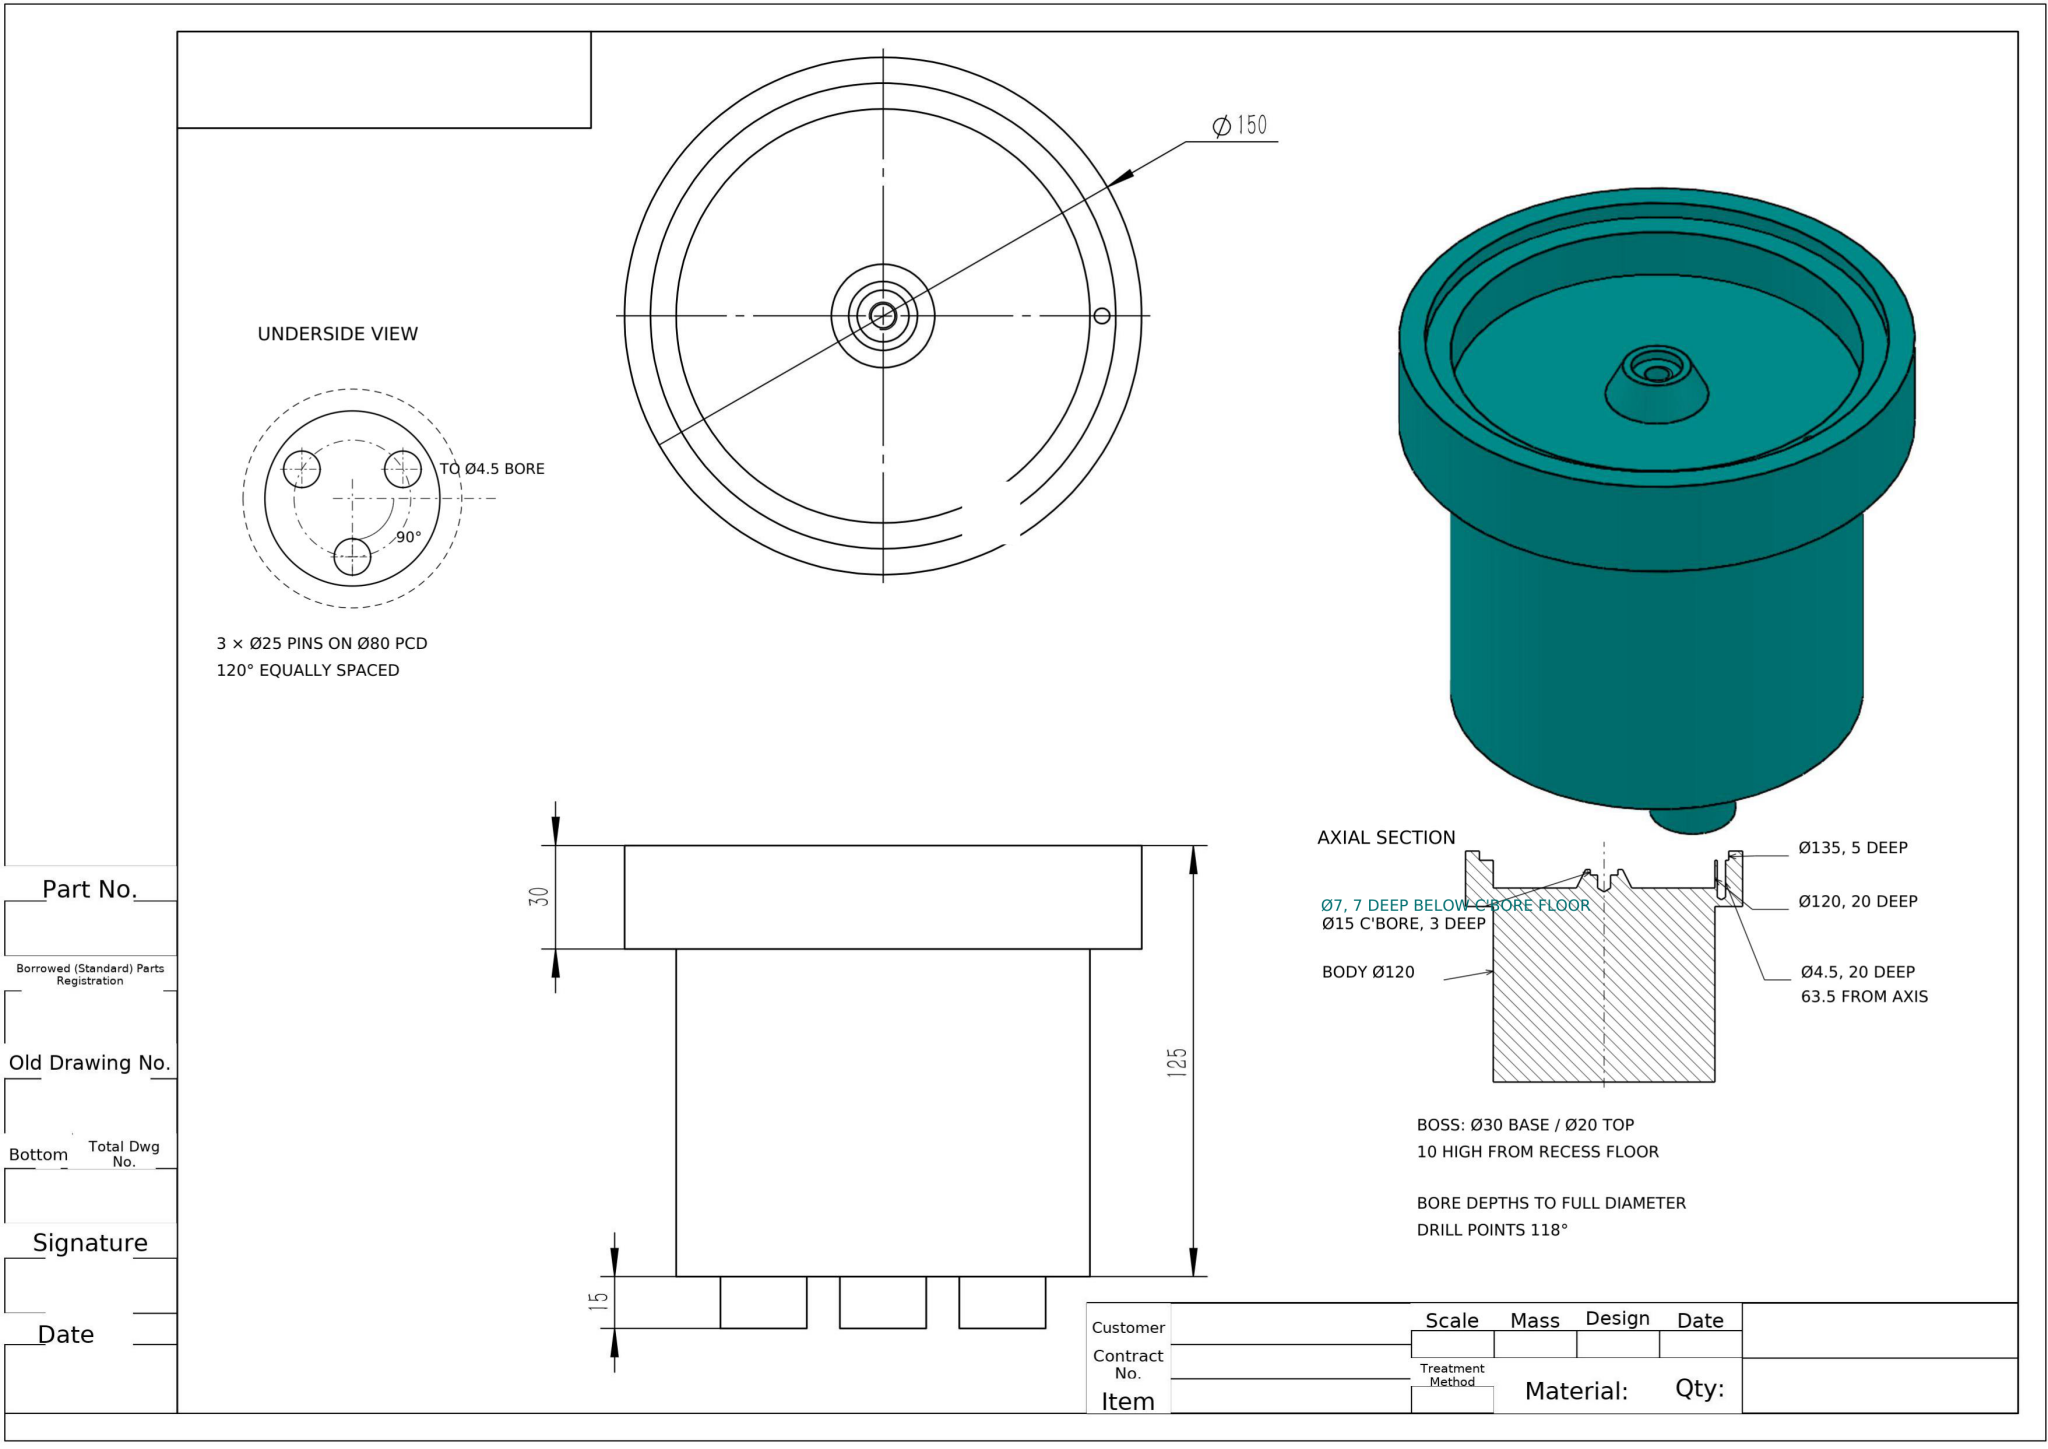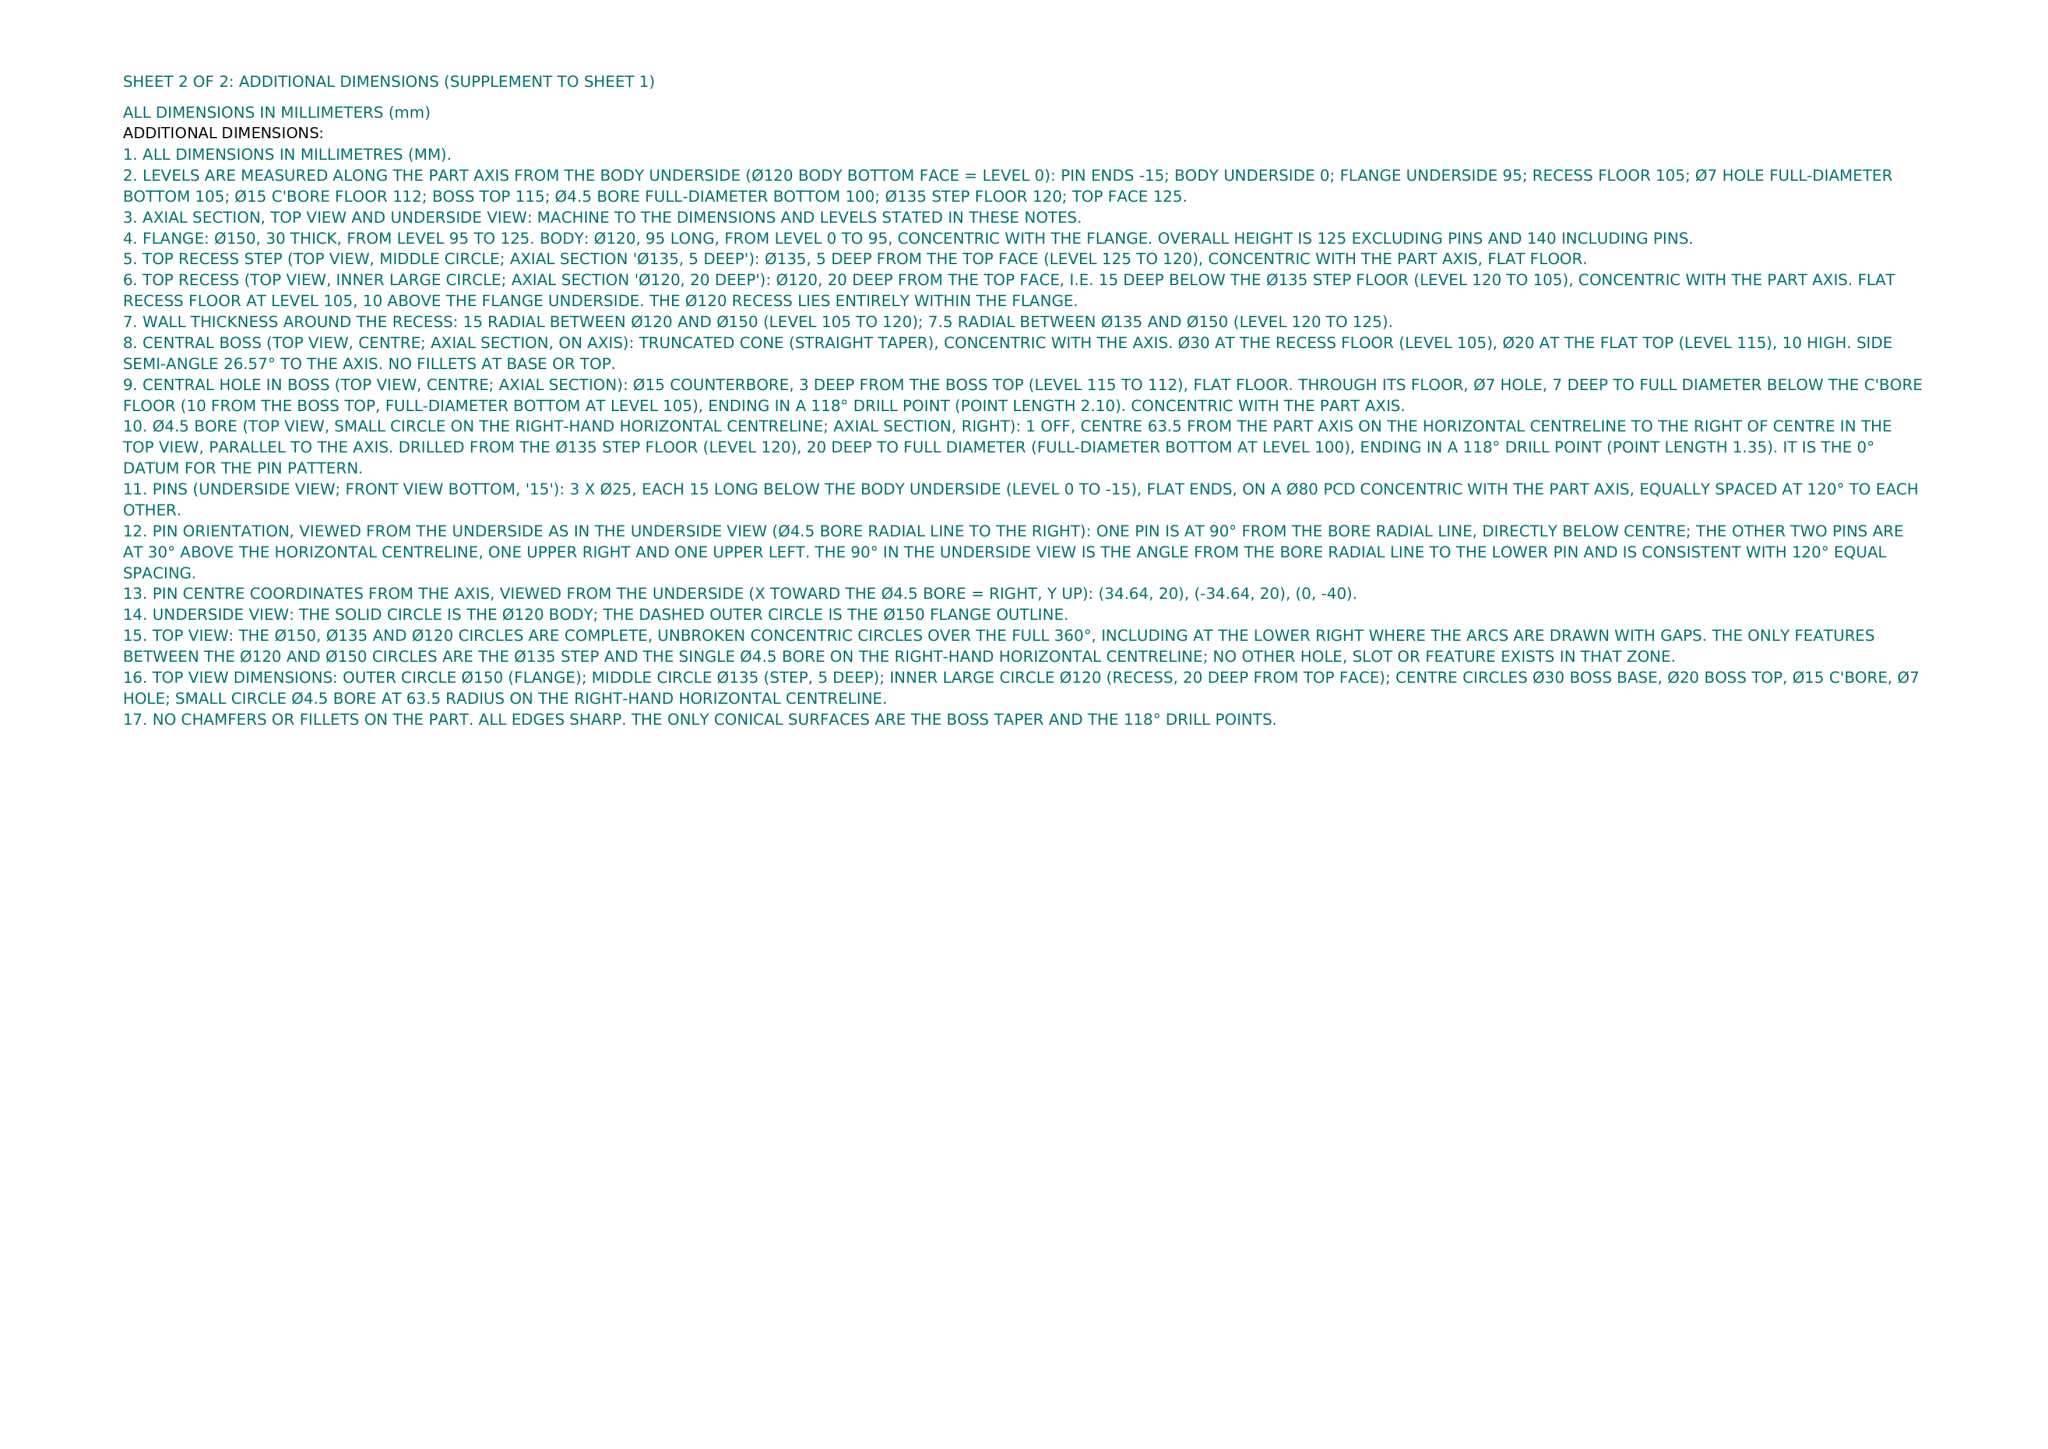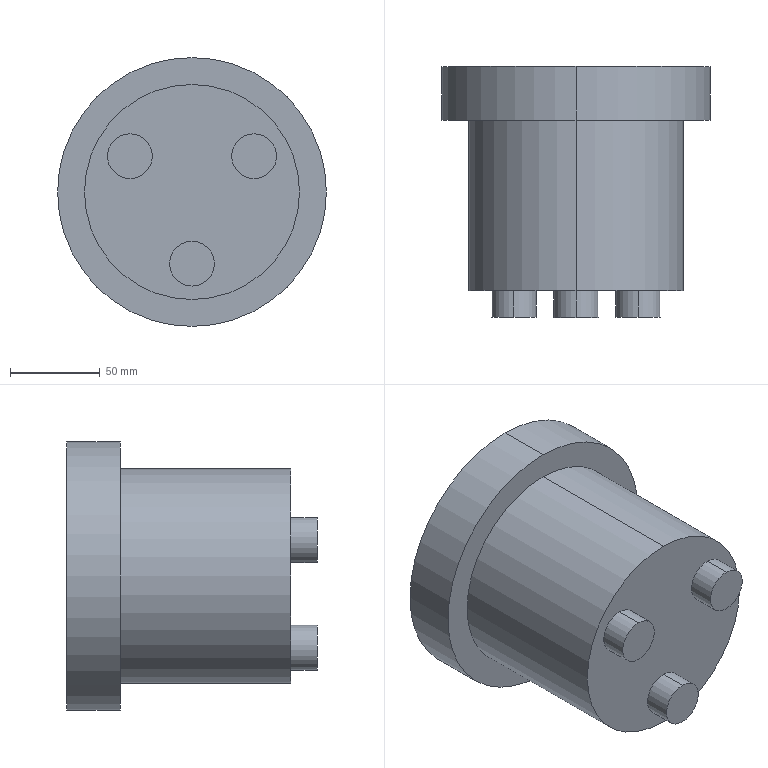Part | NX | mm | 1 solid | 36 faces | box 150 x 140 x 150 mm | volume 1389265 mm3 | cylinder 20 | plane 10 | cone 6 | commonest cylinder face diameters 25 x6 120 x4 4.5 x2 7 x2 15 x2 135 x2 150 x2